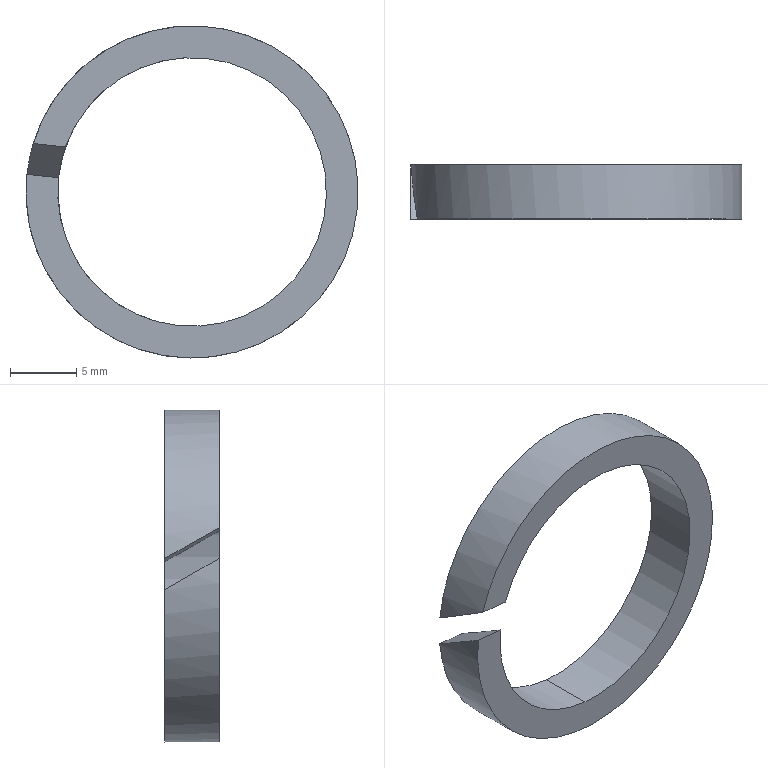Component | SolidWorks | YC1-250-04BalancerAssembly#16673-1_GBSpringWasherM20_GB_FASTENER_WASHER_SW16-1 | 1 solid | 9 faces | box 25.1 x 4.1 x 25.1 mm | volume 678 mm3 | cylinder 5 | plane 4 | commonest cylinder face diameters 20.3 x3 25.1 x2 | material Plain Carbon Steel
STEP:
#1=COLOUR_RGB('',0.7922,0.8196,0.9333);
#2=FILL_AREA_STYLE_COLOUR('',#1);
#3=FILL_AREA_STYLE('',(#2));
#4=SURFACE_STYLE_FILL_AREA(#3);
#5=SURFACE_SIDE_STYLE('',(#4));
#6=SURFACE_STYLE_USAGE(.BOTH.,#5);
#7=PRESENTATION_STYLE_ASSIGNMENT((#6));
#8=CARTESIAN_POINT('',(-13.335,185.039,5.13));
#9=VERTEX_POINT('',#8);
#10=CARTESIAN_POINT('',(-13.42,185.039,4.335));
#11=VERTEX_POINT('',#10);
#12=CARTESIAN_POINT('',(-13.378,185.039,4.733));
#13=DIRECTION('',(-0.,1.,0.));
#14=DIRECTION('',(0.9944,0.,-0.1059));
#15=AXIS2_PLACEMENT_3D('',#12,#13,#14);
#16=CIRCLE('',#15,0.3996);
#17=EDGE_CURVE('',#9,#11,#16,.T.);
#18=ORIENTED_EDGE('',*,*,#17,.F.);
#19=CARTESIAN_POINT('',(-13.335,185.201,5.13));
#20=VERTEX_POINT('',#19);
#21=CARTESIAN_POINT('',(-13.335,185.039,5.13));
#22=DIRECTION('',(-0.,1.,0.));
#23=VECTOR('',#22,39.37);
#24=LINE('',#21,#23);
#25=EDGE_CURVE('',#9,#20,#24,.T.);
#26=ORIENTED_EDGE('',*,*,#25,.T.);
#27=CARTESIAN_POINT('',(-13.42,185.201,4.335));
#28=VERTEX_POINT('',#27);
#29=CARTESIAN_POINT('',(-13.378,185.201,4.733));
#30=DIRECTION('',(-0.,1.,0.));
#31=DIRECTION('',(0.9944,0.,-0.1059));
#32=AXIS2_PLACEMENT_3D('',#29,#30,#31);
#33=CIRCLE('',#32,0.3996);
#34=EDGE_CURVE('',#20,#28,#33,.T.);
#35=ORIENTED_EDGE('',*,*,#34,.T.);
#36=CARTESIAN_POINT('',(-13.42,185.039,4.335));
#37=DIRECTION('',(-0.,1.,0.));
#38=VECTOR('',#37,39.37);
#39=LINE('',#36,#38);
#40=EDGE_CURVE('',#11,#28,#39,.T.);
#41=ORIENTED_EDGE('',*,*,#40,.F.);
#42=EDGE_LOOP('',(#18,#26,#35,#41));
#43=FACE_OUTER_BOUND('',#42,.T.);
#44=CARTESIAN_POINT('',(-13.378,185.039,4.733));
#45=DIRECTION('',(-0.,1.,0.));
#46=DIRECTION('',(-0.1059,0.,-0.9944));
#47=AXIS2_PLACEMENT_3D('',#44,#45,#46);
#48=CYLINDRICAL_SURFACE('',#47,0.3996);
#49=ADVANCED_FACE('',(#43),#48,.F.);
#50=CARTESIAN_POINT('',(-13.775,185.039,4.775));
#51=VERTEX_POINT('',#50);
#52=CARTESIAN_POINT('',(-13.378,185.039,4.733));
#53=DIRECTION('',(-0.,1.,0.));
#54=DIRECTION('',(0.9944,0.,-0.1059));
#55=AXIS2_PLACEMENT_3D('',#52,#53,#54);
#56=CIRCLE('',#55,0.3996);
#57=EDGE_CURVE('',#11,#51,#56,.T.);
#58=ORIENTED_EDGE('',*,*,#57,.F.);
#59=ORIENTED_EDGE('',*,*,#40,.T.);
#60=CARTESIAN_POINT('',(-13.774,185.201,4.681));
#61=VERTEX_POINT('',#60);
#62=CARTESIAN_POINT('',(-13.378,185.201,4.733));
#63=DIRECTION('',(-0.,1.,0.));
#64=DIRECTION('',(0.9944,0.,-0.1059));
#65=AXIS2_PLACEMENT_3D('',#62,#63,#64);
#66=CIRCLE('',#65,0.3996);
#67=EDGE_CURVE('',#28,#61,#66,.T.);
#68=ORIENTED_EDGE('',*,*,#67,.T.);
#69=CARTESIAN_POINT('',(-13.775,185.039,4.775));
#70=CARTESIAN_POINT('',(-13.778,185.094,4.744));
#71=CARTESIAN_POINT('',(-13.778,185.148,4.712));
#72=CARTESIAN_POINT('',(-13.774,185.201,4.681));
#73=(BOUNDED_CURVE()B_SPLINE_CURVE(3,(#69,#70,#71,#72),.UNSPECIFIED.,.F.,.T.)B_SPLINE_CURVE_WITH_KNOTS((4,4),(4.712,4.948),.UNSPECIFIED.)CURVE()GEOMETRIC_REPRESENTATION_ITEM()RATIONAL_B_SPLINE_CURVE((1.,0.9954,0.9954,1.))REPRESENTATION_ITEM(''));
#74=EDGE_CURVE('',#51,#61,#73,.T.);
#75=ORIENTED_EDGE('',*,*,#74,.F.);
#76=EDGE_LOOP('',(#58,#59,#68,#75));
#77=FACE_OUTER_BOUND('',#76,.T.);
#78=CARTESIAN_POINT('',(-13.378,185.039,4.733));
#79=DIRECTION('',(-0.,1.,0.));
#80=DIRECTION('',(-0.1059,0.,-0.9944));
#81=AXIS2_PLACEMENT_3D('',#78,#79,#80);
#82=CYLINDRICAL_SURFACE('',#81,0.3996);
#83=ADVANCED_FACE('',(#77),#82,.F.);
#84=CARTESIAN_POINT('',(-13.87,185.201,4.691));
#85=VERTEX_POINT('',#84);
#86=CARTESIAN_POINT('',(-12.886,185.201,4.68));
#87=VERTEX_POINT('',#86);
#88=CARTESIAN_POINT('',(-13.378,185.201,4.733));
#89=DIRECTION('',(0.,-1.,0.));
#90=DIRECTION('',(0.9944,0.,-0.1059));
#91=AXIS2_PLACEMENT_3D('',#88,#89,#90);
#92=CIRCLE('',#91,0.4941);
#93=EDGE_CURVE('',#85,#87,#92,.T.);
#94=ORIENTED_EDGE('',*,*,#93,.T.);
#95=CARTESIAN_POINT('',(-12.886,185.039,4.68));
#96=VERTEX_POINT('',#95);
#97=CARTESIAN_POINT('',(-12.886,185.201,4.68));
#98=DIRECTION('',(0.,-1.,0.));
#99=VECTOR('',#98,39.37);
#100=LINE('',#97,#99);
#101=EDGE_CURVE('',#87,#96,#100,.T.);
#102=ORIENTED_EDGE('',*,*,#101,.T.);
#103=CARTESIAN_POINT('',(-13.869,185.039,4.785));
#104=VERTEX_POINT('',#103);
#105=CARTESIAN_POINT('',(-13.378,185.039,4.733));
#106=DIRECTION('',(-0.,1.,-0.));
#107=DIRECTION('',(0.9944,0.,-0.1059));
#108=AXIS2_PLACEMENT_3D('',#105,#106,#107);
#109=CIRCLE('',#108,0.4941);
#110=EDGE_CURVE('',#96,#104,#109,.T.);
#111=ORIENTED_EDGE('',*,*,#110,.T.);
#112=CARTESIAN_POINT('',(-13.87,185.201,4.691));
#113=CARTESIAN_POINT('',(-13.873,185.148,4.723));
#114=CARTESIAN_POINT('',(-13.872,185.094,4.754));
#115=CARTESIAN_POINT('',(-13.869,185.039,4.785));
#116=(BOUNDED_CURVE()B_SPLINE_CURVE(3,(#112,#113,#114,#115),.UNSPECIFIED.,.F.,.T.)B_SPLINE_CURVE_WITH_KNOTS((4,4),(4.523,4.712),.UNSPECIFIED.)CURVE()GEOMETRIC_REPRESENTATION_ITEM()RATIONAL_B_SPLINE_CURVE((1.,0.997,0.997,1.))REPRESENTATION_ITEM(''));
#117=EDGE_CURVE('',#85,#104,#116,.T.);
#118=ORIENTED_EDGE('',*,*,#117,.F.);
#119=EDGE_LOOP('',(#94,#102,#111,#118));
#120=FACE_OUTER_BOUND('',#119,.T.);
#121=CARTESIAN_POINT('',(-13.378,185.201,4.733));
#122=DIRECTION('',(0.,-1.,0.));
#123=DIRECTION('',(0.9944,0.,-0.1059));
#124=AXIS2_PLACEMENT_3D('',#121,#122,#123);
#125=CYLINDRICAL_SURFACE('',#124,0.4941);
#126=ADVANCED_FACE('',(#120),#125,.T.);
#127=CARTESIAN_POINT('',(-13.775,185.201,4.775));
#128=VERTEX_POINT('',#127);
#129=CARTESIAN_POINT('',(-13.378,185.201,4.733));
#130=DIRECTION('',(-0.,1.,0.));
#131=DIRECTION('',(0.9944,0.,-0.1059));
#132=AXIS2_PLACEMENT_3D('',#129,#130,#131);
#133=CIRCLE('',#132,0.3996);
#134=EDGE_CURVE('',#128,#20,#133,.T.);
#135=ORIENTED_EDGE('',*,*,#134,.F.);
#136=CARTESIAN_POINT('',(-13.869,185.201,4.785));
#137=VERTEX_POINT('',#136);
#138=CARTESIAN_POINT('',(-13.378,185.201,4.733));
#139=DIRECTION('',(0.9944,0.,-0.1059));
#140=VECTOR('',#139,39.37);
#141=LINE('',#138,#140);
#142=EDGE_CURVE('',#137,#128,#141,.T.);
#143=ORIENTED_EDGE('',*,*,#142,.F.);
#144=CARTESIAN_POINT('',(-13.378,185.201,4.733));
#145=DIRECTION('',(0.,-1.,0.));
#146=DIRECTION('',(0.9944,0.,-0.1059));
#147=AXIS2_PLACEMENT_3D('',#144,#145,#146);
#148=CIRCLE('',#147,0.4941);
#149=EDGE_CURVE('',#87,#137,#148,.T.);
#150=ORIENTED_EDGE('',*,*,#149,.F.);
#151=ORIENTED_EDGE('',*,*,#93,.F.);
#152=CARTESIAN_POINT('',(-13.388,185.201,4.64));
#153=DIRECTION('',(-0.9944,-0.,0.1059));
#154=VECTOR('',#153,39.37);
#155=LINE('',#152,#154);
#156=EDGE_CURVE('',#61,#85,#155,.T.);
#157=ORIENTED_EDGE('',*,*,#156,.F.);
#158=ORIENTED_EDGE('',*,*,#67,.F.);
#159=ORIENTED_EDGE('',*,*,#34,.F.);
#160=EDGE_LOOP('',(#135,#143,#150,#151,#157,#158,#159));
#161=FACE_OUTER_BOUND('',#160,.T.);
#162=CARTESIAN_POINT('',(-13.378,185.201,4.733));
#163=DIRECTION('',(0.,-1.,-0.));
#164=DIRECTION('',(0.9944,0.,-0.1059));
#165=AXIS2_PLACEMENT_3D('',#162,#163,#164);
#166=PLANE('',#165);
#167=ADVANCED_FACE('',(#161),#166,.F.);
#168=CARTESIAN_POINT('',(-13.869,185.039,4.785));
#169=DIRECTION('',(0.9944,0.,-0.1059));
#170=VECTOR('',#169,39.37);
#171=LINE('',#168,#170);
#172=EDGE_CURVE('',#104,#51,#171,.T.);
#173=ORIENTED_EDGE('',*,*,#172,.T.);
#174=ORIENTED_EDGE('',*,*,#74,.T.);
#175=ORIENTED_EDGE('',*,*,#156,.T.);
#176=ORIENTED_EDGE('',*,*,#117,.T.);
#177=EDGE_LOOP('',(#173,#174,#175,#176));
#178=FACE_OUTER_BOUND('',#177,.T.);
#179=CARTESIAN_POINT('',(-13.869,185.039,4.785));
#180=DIRECTION('',(0.0917,0.5,0.8612));
#181=DIRECTION('',(-0.05295,0.866,-0.4972));
#182=AXIS2_PLACEMENT_3D('',#179,#180,#181);
#183=PLANE('',#182);
#184=ADVANCED_FACE('',(#178),#183,.T.);
#185=ORIENTED_EDGE('',*,*,#142,.T.);
#186=CARTESIAN_POINT('',(-13.754,185.039,4.866));
#187=VERTEX_POINT('',#186);
#188=CARTESIAN_POINT('',(-13.775,185.201,4.775));
#189=CARTESIAN_POINT('',(-13.772,185.146,4.806));
#190=CARTESIAN_POINT('',(-13.765,185.092,4.837));
#191=CARTESIAN_POINT('',(-13.754,185.039,4.866));
#192=(BOUNDED_CURVE()B_SPLINE_CURVE(3,(#188,#189,#190,#191),.UNSPECIFIED.,.F.,.T.)B_SPLINE_CURVE_WITH_KNOTS((4,4),(1.571,1.806),.UNSPECIFIED.)CURVE()GEOMETRIC_REPRESENTATION_ITEM()RATIONAL_B_SPLINE_CURVE((1.,0.9954,0.9954,1.))REPRESENTATION_ITEM(''));
#193=EDGE_CURVE('',#128,#187,#192,.T.);
#194=ORIENTED_EDGE('',*,*,#193,.T.);
#195=CARTESIAN_POINT('',(-13.85,185.039,4.877));
#196=VERTEX_POINT('',#195);
#197=CARTESIAN_POINT('',(-13.859,185.039,4.878));
#198=DIRECTION('',(-0.9944,-0.,0.1059));
#199=VECTOR('',#198,39.37);
#200=LINE('',#197,#199);
#201=EDGE_CURVE('',#187,#196,#200,.T.);
#202=ORIENTED_EDGE('',*,*,#201,.T.);
#203=CARTESIAN_POINT('',(-13.85,185.039,4.877));
#204=CARTESIAN_POINT('',(-13.859,185.093,4.847));
#205=CARTESIAN_POINT('',(-13.866,185.147,4.816));
#206=CARTESIAN_POINT('',(-13.869,185.201,4.785));
#207=(BOUNDED_CURVE()B_SPLINE_CURVE(3,(#203,#204,#205,#206),.UNSPECIFIED.,.F.,.T.)B_SPLINE_CURVE_WITH_KNOTS((4,4),(1.381,1.571),.UNSPECIFIED.)CURVE()GEOMETRIC_REPRESENTATION_ITEM()RATIONAL_B_SPLINE_CURVE((1.,0.997,0.997,1.))REPRESENTATION_ITEM(''));
#208=EDGE_CURVE('',#196,#137,#207,.T.);
#209=ORIENTED_EDGE('',*,*,#208,.T.);
#210=EDGE_LOOP('',(#185,#194,#202,#209));
#211=FACE_OUTER_BOUND('',#210,.T.);
#212=CARTESIAN_POINT('',(-13.869,185.201,4.785));
#213=DIRECTION('',(-0.0917,-0.5,-0.8612));
#214=DIRECTION('',(0.05295,-0.866,0.4972));
#215=AXIS2_PLACEMENT_3D('',#212,#213,#214);
#216=PLANE('',#215);
#217=ADVANCED_FACE('',(#211),#216,.T.);
#218=ORIENTED_EDGE('',*,*,#101,.F.);
#219=ORIENTED_EDGE('',*,*,#149,.T.);
#220=ORIENTED_EDGE('',*,*,#208,.F.);
#221=CARTESIAN_POINT('',(-13.378,185.039,4.733));
#222=DIRECTION('',(-0.,1.,-0.));
#223=DIRECTION('',(0.9944,0.,-0.1059));
#224=AXIS2_PLACEMENT_3D('',#221,#222,#223);
#225=CIRCLE('',#224,0.4941);
#226=EDGE_CURVE('',#196,#96,#225,.T.);
#227=ORIENTED_EDGE('',*,*,#226,.T.);
#228=EDGE_LOOP('',(#218,#219,#220,#227));
#229=FACE_OUTER_BOUND('',#228,.T.);
#230=CARTESIAN_POINT('',(-13.378,185.201,4.733));
#231=DIRECTION('',(0.,-1.,0.));
#232=DIRECTION('',(0.9944,0.,-0.1059));
#233=AXIS2_PLACEMENT_3D('',#230,#231,#232);
#234=CYLINDRICAL_SURFACE('',#233,0.4941);
#235=ADVANCED_FACE('',(#229),#234,.T.);
#236=ORIENTED_EDGE('',*,*,#201,.F.);
#237=CARTESIAN_POINT('',(-13.378,185.039,4.733));
#238=DIRECTION('',(-0.,1.,0.));
#239=DIRECTION('',(0.9944,0.,-0.1059));
#240=AXIS2_PLACEMENT_3D('',#237,#238,#239);
#241=CIRCLE('',#240,0.3996);
#242=EDGE_CURVE('',#187,#9,#241,.T.);
#243=ORIENTED_EDGE('',*,*,#242,.T.);
#244=ORIENTED_EDGE('',*,*,#17,.T.);
#245=ORIENTED_EDGE('',*,*,#57,.T.);
#246=ORIENTED_EDGE('',*,*,#172,.F.);
#247=ORIENTED_EDGE('',*,*,#110,.F.);
#248=ORIENTED_EDGE('',*,*,#226,.F.);
#249=EDGE_LOOP('',(#236,#243,#244,#245,#246,#247,#248));
#250=FACE_OUTER_BOUND('',#249,.T.);
#251=CARTESIAN_POINT('',(-13.378,185.039,4.733));
#252=DIRECTION('',(0.,-1.,-0.));
#253=DIRECTION('',(0.9944,0.,-0.1059));
#254=AXIS2_PLACEMENT_3D('',#251,#252,#253);
#255=PLANE('',#254);
#256=ADVANCED_FACE('',(#250),#255,.T.);
#257=ORIENTED_EDGE('',*,*,#25,.F.);
#258=ORIENTED_EDGE('',*,*,#242,.F.);
#259=ORIENTED_EDGE('',*,*,#193,.F.);
#260=ORIENTED_EDGE('',*,*,#134,.T.);
#261=EDGE_LOOP('',(#257,#258,#259,#260));
#262=FACE_OUTER_BOUND('',#261,.T.);
#263=CARTESIAN_POINT('',(-13.378,185.039,4.733));
#264=DIRECTION('',(-0.,1.,0.));
#265=DIRECTION('',(-0.1059,0.,-0.9944));
#266=AXIS2_PLACEMENT_3D('',#263,#264,#265);
#267=CYLINDRICAL_SURFACE('',#266,0.3996);
#268=ADVANCED_FACE('',(#262),#267,.F.);
#269=CLOSED_SHELL('',(#49,#83,#126,#167,#184,#217,#235,#256,#268));
#270=MANIFOLD_SOLID_BREP('',#269);
#271=STYLED_ITEM('',(#7),#270);
#272=(LENGTH_UNIT()NAMED_UNIT(*)SI_UNIT($,.METRE.));
#273=LENGTH_MEASURE_WITH_UNIT(LENGTH_MEASURE(0.0254),#272);
#274=DIMENSIONAL_EXPONENTS(1.,0.,0.,0.,0.,0.,0.);
#275=(CONVERSION_BASED_UNIT('',#273)LENGTH_UNIT()NAMED_UNIT(#274));
#276=UNCERTAINTY_MEASURE_WITH_UNIT(LENGTH_MEASURE(0.00001),#275,'','');
#277=(NAMED_UNIT(*)PLANE_ANGLE_UNIT()SI_UNIT($,.RADIAN.));
#278=(NAMED_UNIT(*)SI_UNIT($,.STERADIAN.)SOLID_ANGLE_UNIT());
#279=(GEOMETRIC_REPRESENTATION_CONTEXT(3)GLOBAL_UNCERTAINTY_ASSIGNED_CONTEXT((#276))GLOBAL_UNIT_ASSIGNED_CONTEXT((#275,#277,#278))REPRESENTATION_CONTEXT('',''));
#280=MECHANICAL_DESIGN_GEOMETRIC_PRESENTATION_REPRESENTATION('',(#271),#279);
#281=PRESENTATION_LAYER_ASSIGNMENT('','',(#271));
#282=CARTESIAN_POINT('',(0.,0.,0.));
#283=DIRECTION('',(0.,0.,1.));
#284=DIRECTION('',(1.,0.,0.));
#285=AXIS2_PLACEMENT_3D('',#282,#283,#284);
#286=(LENGTH_UNIT()NAMED_UNIT(*)SI_UNIT($,.METRE.));
#287=LENGTH_MEASURE_WITH_UNIT(LENGTH_MEASURE(0.0254),#286);
#288=DIMENSIONAL_EXPONENTS(1.,0.,0.,0.,0.,0.,0.);
#289=(CONVERSION_BASED_UNIT('',#287)LENGTH_UNIT()NAMED_UNIT(#288));
#290=UNCERTAINTY_MEASURE_WITH_UNIT(LENGTH_MEASURE(0.00001),#289,'','');
#291=(NAMED_UNIT(*)PLANE_ANGLE_UNIT()SI_UNIT($,.RADIAN.));
#292=(NAMED_UNIT(*)SI_UNIT($,.STERADIAN.)SOLID_ANGLE_UNIT());
#293=(GEOMETRIC_REPRESENTATION_CONTEXT(3)GLOBAL_UNCERTAINTY_ASSIGNED_CONTEXT((#290))GLOBAL_UNIT_ASSIGNED_CONTEXT((#289,#291,#292))REPRESENTATION_CONTEXT('',''));
#294=ADVANCED_BREP_SHAPE_REPRESENTATION('',(#270,#285),#293);